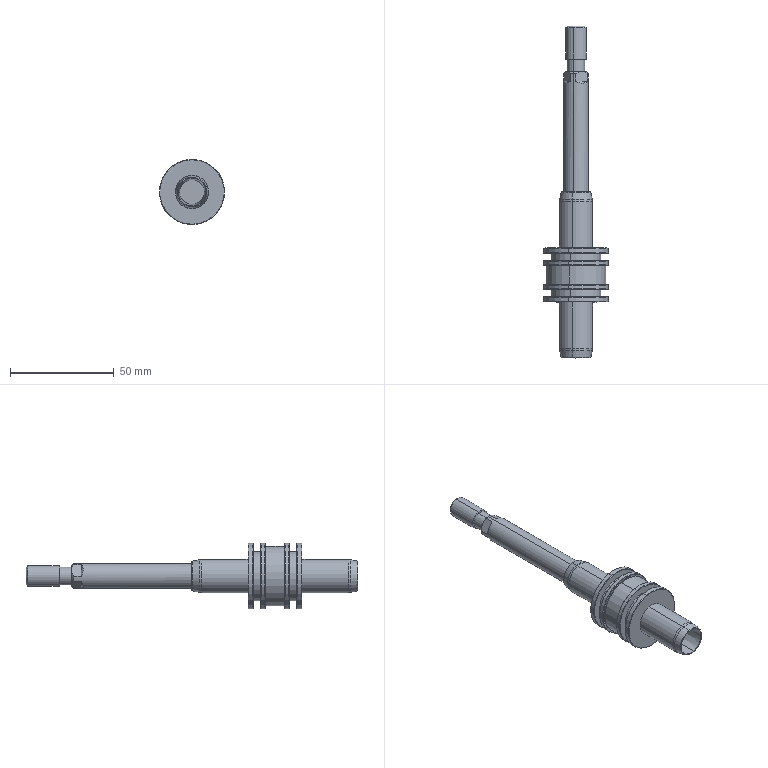Component | SolidWorks | HZ022-SE32x25S-1_HZ022-SE32x25S (3)-1 | 1 solid | 89 faces | volume 30125 mm3 | cone 31 | cylinder 24 | plane 22 | spline 12 | commonest cylinder face diameters 31.5 x8 16 x4 24 x4 10 x2 8.6 x2 12 x2 28.9 x2 | material AL6061